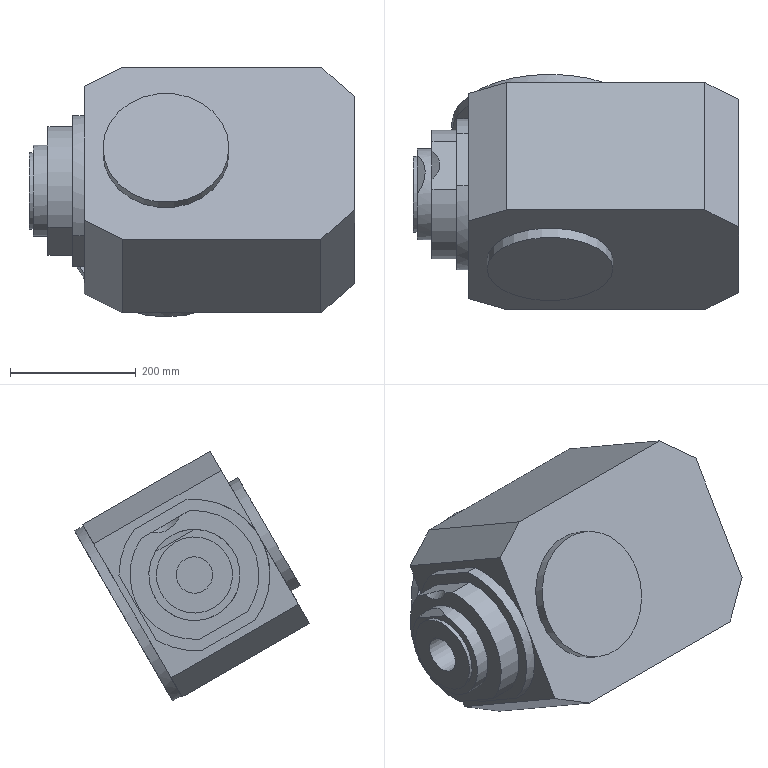Component | NX | SIM15_B1_ACHSE | 1 solid | 37 faces | volume 34597758 mm3 | plane 25 | cylinder 12 | commonest cylinder face diameters 240 x3 205 x2 145 x1 121 x1 100 x1 312 x1 200 x1 58 x1